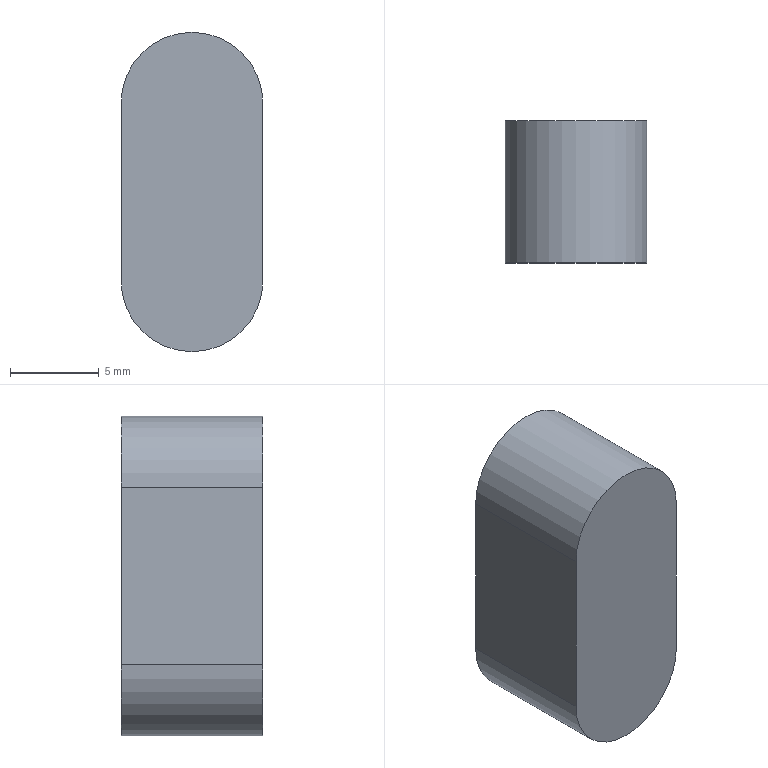Component | NX | FLAT_KEY_3 | 1 solid | 6 faces | box 8 x 8 x 18 mm | volume 1042 mm3 | plane 4 | cylinder 2 | commonest cylinder face diameters 8 x2
STEP:
#1=CARTESIAN_POINT('',(0.,0.,0.));
#2=DIRECTION('',(0.,0.,1.));
#3=DIRECTION('',(1.,0.,0.));
#4=AXIS2_PLACEMENT_3D('',#1,#2,#3);
#5=CARTESIAN_POINT('',(-602.175,316.681,-695.));
#6=VERTEX_POINT('',#5);
#7=CARTESIAN_POINT('',(-602.175,316.681,-685.));
#8=VERTEX_POINT('',#7);
#9=CARTESIAN_POINT('',(-602.175,316.681,-690.));
#10=DIRECTION('',(0.,0.,1.));
#11=VECTOR('',#10,1.);
#12=LINE('',#9,#11);
#13=CARTESIAN_POINT('',(-598.175,316.681,-690.));
#14=DIRECTION('',(0.,-1.,0.));
#15=DIRECTION('',(0.,0.,-1.));
#16=AXIS2_PLACEMENT_3D('',#13,#14,#15);
#17=PLANE('',#16);
#18=CARTESIAN_POINT('',(0.,-4.));
#19=DIRECTION('',(-1.,0.));
#20=VECTOR('',#19,1.);
#21=LINE('',#18,#20);
#22=(GEOMETRIC_REPRESENTATION_CONTEXT(2)PARAMETRIC_REPRESENTATION_CONTEXT()REPRESENTATION_CONTEXT('',''));
#23=DEFINITIONAL_REPRESENTATION('',(#21),#22);
#24=PCURVE('',#17,#23);
#25=CARTESIAN_POINT('',(-602.175,324.681,-690.));
#26=DIRECTION('',(-1.,0.,0.));
#27=DIRECTION('',(0.,1.,0.));
#28=AXIS2_PLACEMENT_3D('',#25,#26,#27);
#29=PLANE('',#28);
#30=CARTESIAN_POINT('',(-8.,0.));
#31=DIRECTION('',(0.,-1.));
#32=VECTOR('',#31,1.);
#33=LINE('',#30,#32);
#34=(GEOMETRIC_REPRESENTATION_CONTEXT(2)PARAMETRIC_REPRESENTATION_CONTEXT()REPRESENTATION_CONTEXT('',''));
#35=DEFINITIONAL_REPRESENTATION('',(#33),#34);
#36=PCURVE('',#29,#35);
#37=SURFACE_CURVE('',#12,(#24,#36),.PCURVE_S1.);
#38=EDGE_CURVE('',#6,#8,#37,.T.);
#39=ORIENTED_EDGE('',*,*,#38,.F.);
#40=CARTESIAN_POINT('',(-594.175,316.681,-695.));
#41=VERTEX_POINT('',#40);
#42=CARTESIAN_POINT('',(-598.175,316.681,-695.));
#43=DIRECTION('',(0.,-1.,0.));
#44=DIRECTION('',(0.,0.,-1.));
#45=AXIS2_PLACEMENT_3D('',#42,#43,#44);
#46=CIRCLE('',#45,4.);
#47=CARTESIAN_POINT('',(5.,0.));
#48=DIRECTION('',(1.,0.));
#49=AXIS2_PLACEMENT_2D('',#47,#48);
#50=CIRCLE('',#49,4.);
#51=(GEOMETRIC_REPRESENTATION_CONTEXT(2)PARAMETRIC_REPRESENTATION_CONTEXT()REPRESENTATION_CONTEXT('',''));
#52=DEFINITIONAL_REPRESENTATION('',(#50),#51);
#53=PCURVE('',#17,#52);
#54=CARTESIAN_POINT('',(-598.175,324.681,-695.));
#55=DIRECTION('',(0.,-1.,0.));
#56=DIRECTION('',(0.,0.,-1.));
#57=AXIS2_PLACEMENT_3D('',#54,#55,#56);
#58=CYLINDRICAL_SURFACE('',#57,4.);
#59=CARTESIAN_POINT('',(0.,8.));
#60=DIRECTION('',(1.,0.));
#61=VECTOR('',#60,1.);
#62=LINE('',#59,#61);
#63=(GEOMETRIC_REPRESENTATION_CONTEXT(2)PARAMETRIC_REPRESENTATION_CONTEXT()REPRESENTATION_CONTEXT('',''));
#64=DEFINITIONAL_REPRESENTATION('',(#62),#63);
#65=PCURVE('',#58,#64);
#66=SURFACE_CURVE('',#46,(#53,#65),.PCURVE_S1.);
#67=EDGE_CURVE('',#6,#41,#66,.T.);
#68=ORIENTED_EDGE('',*,*,#67,.T.);
#69=CARTESIAN_POINT('',(-594.175,316.681,-685.));
#70=VERTEX_POINT('',#69);
#71=CARTESIAN_POINT('',(-594.175,316.681,-690.));
#72=DIRECTION('',(0.,0.,-1.));
#73=VECTOR('',#72,1.);
#74=LINE('',#71,#73);
#75=CARTESIAN_POINT('',(0.,4.));
#76=DIRECTION('',(1.,0.));
#77=VECTOR('',#76,1.);
#78=LINE('',#75,#77);
#79=(GEOMETRIC_REPRESENTATION_CONTEXT(2)PARAMETRIC_REPRESENTATION_CONTEXT()REPRESENTATION_CONTEXT('',''));
#80=DEFINITIONAL_REPRESENTATION('',(#78),#79);
#81=PCURVE('',#17,#80);
#82=CARTESIAN_POINT('',(-594.175,324.681,-690.));
#83=DIRECTION('',(1.,0.,0.));
#84=DIRECTION('',(0.,-1.,0.));
#85=AXIS2_PLACEMENT_3D('',#82,#83,#84);
#86=PLANE('',#85);
#87=CARTESIAN_POINT('',(8.,0.));
#88=DIRECTION('',(0.,1.));
#89=VECTOR('',#88,1.);
#90=LINE('',#87,#89);
#91=(GEOMETRIC_REPRESENTATION_CONTEXT(2)PARAMETRIC_REPRESENTATION_CONTEXT()REPRESENTATION_CONTEXT('',''));
#92=DEFINITIONAL_REPRESENTATION('',(#90),#91);
#93=PCURVE('',#86,#92);
#94=SURFACE_CURVE('',#74,(#81,#93),.PCURVE_S1.);
#95=EDGE_CURVE('',#70,#41,#94,.T.);
#96=ORIENTED_EDGE('',*,*,#95,.F.);
#97=CARTESIAN_POINT('',(-598.175,316.681,-685.));
#98=DIRECTION('',(0.,-1.,0.));
#99=DIRECTION('',(0.,0.,-1.));
#100=AXIS2_PLACEMENT_3D('',#97,#98,#99);
#101=CIRCLE('',#100,4.);
#102=CARTESIAN_POINT('',(-5.,0.));
#103=DIRECTION('',(1.,0.));
#104=AXIS2_PLACEMENT_2D('',#102,#103);
#105=CIRCLE('',#104,4.);
#106=(GEOMETRIC_REPRESENTATION_CONTEXT(2)PARAMETRIC_REPRESENTATION_CONTEXT()REPRESENTATION_CONTEXT('',''));
#107=DEFINITIONAL_REPRESENTATION('',(#105),#106);
#108=PCURVE('',#17,#107);
#109=CARTESIAN_POINT('',(-598.175,324.681,-685.));
#110=DIRECTION('',(0.,-1.,0.));
#111=DIRECTION('',(0.,0.,-1.));
#112=AXIS2_PLACEMENT_3D('',#109,#110,#111);
#113=CYLINDRICAL_SURFACE('',#112,4.);
#114=CARTESIAN_POINT('',(0.,8.));
#115=DIRECTION('',(1.,0.));
#116=VECTOR('',#115,1.);
#117=LINE('',#114,#116);
#118=(GEOMETRIC_REPRESENTATION_CONTEXT(2)PARAMETRIC_REPRESENTATION_CONTEXT()REPRESENTATION_CONTEXT('',''));
#119=DEFINITIONAL_REPRESENTATION('',(#117),#118);
#120=PCURVE('',#113,#119);
#121=SURFACE_CURVE('',#101,(#108,#120),.PCURVE_S1.);
#122=EDGE_CURVE('',#70,#8,#121,.T.);
#123=ORIENTED_EDGE('',*,*,#122,.T.);
#124=EDGE_LOOP('',(#39,#68,#96,#123));
#125=FACE_BOUND('',#124,.T.);
#126=ADVANCED_FACE('',(#125),#17,.T.);
#127=CARTESIAN_POINT('',(-602.175,324.681,-685.));
#128=VERTEX_POINT('',#127);
#129=CARTESIAN_POINT('',(-602.175,324.681,-695.));
#130=VERTEX_POINT('',#129);
#131=CARTESIAN_POINT('',(-602.175,324.681,-690.));
#132=DIRECTION('',(0.,0.,-1.));
#133=VECTOR('',#132,1.);
#134=LINE('',#131,#133);
#135=CARTESIAN_POINT('',(0.,0.));
#136=DIRECTION('',(0.,1.));
#137=VECTOR('',#136,1.);
#138=LINE('',#135,#137);
#139=(GEOMETRIC_REPRESENTATION_CONTEXT(2)PARAMETRIC_REPRESENTATION_CONTEXT()REPRESENTATION_CONTEXT('',''));
#140=DEFINITIONAL_REPRESENTATION('',(#138),#139);
#141=PCURVE('',#29,#140);
#142=CARTESIAN_POINT('',(-598.175,324.681,-690.));
#143=DIRECTION('',(0.,1.,0.));
#144=DIRECTION('',(0.,0.,1.));
#145=AXIS2_PLACEMENT_3D('',#142,#143,#144);
#146=PLANE('',#145);
#147=CARTESIAN_POINT('',(0.,-4.));
#148=DIRECTION('',(-1.,0.));
#149=VECTOR('',#148,1.);
#150=LINE('',#147,#149);
#151=(GEOMETRIC_REPRESENTATION_CONTEXT(2)PARAMETRIC_REPRESENTATION_CONTEXT()REPRESENTATION_CONTEXT('',''));
#152=DEFINITIONAL_REPRESENTATION('',(#150),#151);
#153=PCURVE('',#146,#152);
#154=SURFACE_CURVE('',#134,(#141,#153),.PCURVE_S1.);
#155=EDGE_CURVE('',#128,#130,#154,.T.);
#156=ORIENTED_EDGE('',*,*,#155,.T.);
#157=CARTESIAN_POINT('',(-602.175,324.681,-695.));
#158=DIRECTION('',(0.,-1.,0.));
#159=VECTOR('',#158,1.);
#160=LINE('',#157,#159);
#161=CARTESIAN_POINT('',(0.,5.));
#162=DIRECTION('',(-1.,0.));
#163=VECTOR('',#162,1.);
#164=LINE('',#161,#163);
#165=(GEOMETRIC_REPRESENTATION_CONTEXT(2)PARAMETRIC_REPRESENTATION_CONTEXT()REPRESENTATION_CONTEXT('',''));
#166=DEFINITIONAL_REPRESENTATION('',(#164),#165);
#167=PCURVE('',#29,#166);
#168=CARTESIAN_POINT('',(4.712,0.));
#169=DIRECTION('',(0.,1.));
#170=VECTOR('',#169,1.);
#171=LINE('',#168,#170);
#172=(GEOMETRIC_REPRESENTATION_CONTEXT(2)PARAMETRIC_REPRESENTATION_CONTEXT()REPRESENTATION_CONTEXT('',''));
#173=DEFINITIONAL_REPRESENTATION('',(#171),#172);
#174=PCURVE('',#58,#173);
#175=SURFACE_CURVE('',#160,(#167,#174),.PCURVE_S1.);
#176=EDGE_CURVE('',#130,#6,#175,.T.);
#177=ORIENTED_EDGE('',*,*,#176,.T.);
#178=ORIENTED_EDGE('',*,*,#38,.T.);
#179=CARTESIAN_POINT('',(-602.175,324.681,-685.));
#180=DIRECTION('',(0.,1.,0.));
#181=VECTOR('',#180,1.);
#182=LINE('',#179,#181);
#183=CARTESIAN_POINT('',(0.,-5.));
#184=DIRECTION('',(1.,0.));
#185=VECTOR('',#184,1.);
#186=LINE('',#183,#185);
#187=(GEOMETRIC_REPRESENTATION_CONTEXT(2)PARAMETRIC_REPRESENTATION_CONTEXT()REPRESENTATION_CONTEXT('',''));
#188=DEFINITIONAL_REPRESENTATION('',(#186),#187);
#189=PCURVE('',#29,#188);
#190=CARTESIAN_POINT('',(4.712,0.));
#191=DIRECTION('',(0.,-1.));
#192=VECTOR('',#191,1.);
#193=LINE('',#190,#192);
#194=(GEOMETRIC_REPRESENTATION_CONTEXT(2)PARAMETRIC_REPRESENTATION_CONTEXT()REPRESENTATION_CONTEXT('',''));
#195=DEFINITIONAL_REPRESENTATION('',(#193),#194);
#196=PCURVE('',#113,#195);
#197=SURFACE_CURVE('',#182,(#189,#196),.PCURVE_S1.);
#198=EDGE_CURVE('',#8,#128,#197,.T.);
#199=ORIENTED_EDGE('',*,*,#198,.T.);
#200=EDGE_LOOP('',(#156,#177,#178,#199));
#201=FACE_BOUND('',#200,.T.);
#202=ADVANCED_FACE('',(#201),#29,.T.);
#203=ORIENTED_EDGE('',*,*,#95,.T.);
#204=CARTESIAN_POINT('',(-594.175,324.681,-695.));
#205=VERTEX_POINT('',#204);
#206=CARTESIAN_POINT('',(-594.175,324.681,-695.));
#207=DIRECTION('',(0.,1.,0.));
#208=VECTOR('',#207,1.);
#209=LINE('',#206,#208);
#210=CARTESIAN_POINT('',(0.,5.));
#211=DIRECTION('',(-1.,0.));
#212=VECTOR('',#211,1.);
#213=LINE('',#210,#212);
#214=(GEOMETRIC_REPRESENTATION_CONTEXT(2)PARAMETRIC_REPRESENTATION_CONTEXT()REPRESENTATION_CONTEXT('',''));
#215=DEFINITIONAL_REPRESENTATION('',(#213),#214);
#216=PCURVE('',#86,#215);
#217=CARTESIAN_POINT('',(7.854,0.));
#218=DIRECTION('',(0.,-1.));
#219=VECTOR('',#218,1.);
#220=LINE('',#217,#219);
#221=(GEOMETRIC_REPRESENTATION_CONTEXT(2)PARAMETRIC_REPRESENTATION_CONTEXT()REPRESENTATION_CONTEXT('',''));
#222=DEFINITIONAL_REPRESENTATION('',(#220),#221);
#223=PCURVE('',#58,#222);
#224=SURFACE_CURVE('',#209,(#216,#223),.PCURVE_S1.);
#225=EDGE_CURVE('',#41,#205,#224,.T.);
#226=ORIENTED_EDGE('',*,*,#225,.T.);
#227=CARTESIAN_POINT('',(-594.175,324.681,-685.));
#228=VERTEX_POINT('',#227);
#229=CARTESIAN_POINT('',(-594.175,324.681,-690.));
#230=DIRECTION('',(0.,0.,1.));
#231=VECTOR('',#230,1.);
#232=LINE('',#229,#231);
#233=CARTESIAN_POINT('',(0.,0.));
#234=DIRECTION('',(0.,-1.));
#235=VECTOR('',#234,1.);
#236=LINE('',#233,#235);
#237=(GEOMETRIC_REPRESENTATION_CONTEXT(2)PARAMETRIC_REPRESENTATION_CONTEXT()REPRESENTATION_CONTEXT('',''));
#238=DEFINITIONAL_REPRESENTATION('',(#236),#237);
#239=PCURVE('',#86,#238);
#240=CARTESIAN_POINT('',(0.,4.));
#241=DIRECTION('',(1.,0.));
#242=VECTOR('',#241,1.);
#243=LINE('',#240,#242);
#244=(GEOMETRIC_REPRESENTATION_CONTEXT(2)PARAMETRIC_REPRESENTATION_CONTEXT()REPRESENTATION_CONTEXT('',''));
#245=DEFINITIONAL_REPRESENTATION('',(#243),#244);
#246=PCURVE('',#146,#245);
#247=SURFACE_CURVE('',#232,(#239,#246),.PCURVE_S1.);
#248=EDGE_CURVE('',#205,#228,#247,.T.);
#249=ORIENTED_EDGE('',*,*,#248,.T.);
#250=CARTESIAN_POINT('',(-594.175,324.681,-685.));
#251=DIRECTION('',(0.,-1.,0.));
#252=VECTOR('',#251,1.);
#253=LINE('',#250,#252);
#254=CARTESIAN_POINT('',(0.,-5.));
#255=DIRECTION('',(1.,0.));
#256=VECTOR('',#255,1.);
#257=LINE('',#254,#256);
#258=(GEOMETRIC_REPRESENTATION_CONTEXT(2)PARAMETRIC_REPRESENTATION_CONTEXT()REPRESENTATION_CONTEXT('',''));
#259=DEFINITIONAL_REPRESENTATION('',(#257),#258);
#260=PCURVE('',#86,#259);
#261=CARTESIAN_POINT('',(1.571,0.));
#262=DIRECTION('',(0.,1.));
#263=VECTOR('',#262,1.);
#264=LINE('',#261,#263);
#265=(GEOMETRIC_REPRESENTATION_CONTEXT(2)PARAMETRIC_REPRESENTATION_CONTEXT()REPRESENTATION_CONTEXT('',''));
#266=DEFINITIONAL_REPRESENTATION('',(#264),#265);
#267=PCURVE('',#113,#266);
#268=SURFACE_CURVE('',#253,(#260,#267),.PCURVE_S1.);
#269=EDGE_CURVE('',#228,#70,#268,.T.);
#270=ORIENTED_EDGE('',*,*,#269,.T.);
#271=EDGE_LOOP('',(#203,#226,#249,#270));
#272=FACE_BOUND('',#271,.T.);
#273=ADVANCED_FACE('',(#272),#86,.T.);
#274=CARTESIAN_POINT('',(-598.175,324.681,-695.));
#275=DIRECTION('',(0.,1.,0.));
#276=DIRECTION('',(0.,0.,1.));
#277=AXIS2_PLACEMENT_3D('',#274,#275,#276);
#278=CIRCLE('',#277,4.);
#279=CARTESIAN_POINT('',(-5.,0.));
#280=DIRECTION('',(1.,0.));
#281=AXIS2_PLACEMENT_2D('',#279,#280);
#282=CIRCLE('',#281,4.);
#283=(GEOMETRIC_REPRESENTATION_CONTEXT(2)PARAMETRIC_REPRESENTATION_CONTEXT()REPRESENTATION_CONTEXT('',''));
#284=DEFINITIONAL_REPRESENTATION('',(#282),#283);
#285=PCURVE('',#146,#284);
#286=CARTESIAN_POINT('',(9.425,0.));
#287=DIRECTION('',(-1.,0.));
#288=VECTOR('',#287,1.);
#289=LINE('',#286,#288);
#290=(GEOMETRIC_REPRESENTATION_CONTEXT(2)PARAMETRIC_REPRESENTATION_CONTEXT()REPRESENTATION_CONTEXT('',''));
#291=DEFINITIONAL_REPRESENTATION('',(#289),#290);
#292=PCURVE('',#58,#291);
#293=SURFACE_CURVE('',#278,(#285,#292),.PCURVE_S1.);
#294=EDGE_CURVE('',#205,#130,#293,.T.);
#295=ORIENTED_EDGE('',*,*,#294,.T.);
#296=ORIENTED_EDGE('',*,*,#155,.F.);
#297=CARTESIAN_POINT('',(-598.175,324.681,-685.));
#298=DIRECTION('',(0.,1.,0.));
#299=DIRECTION('',(0.,0.,1.));
#300=AXIS2_PLACEMENT_3D('',#297,#298,#299);
#301=CIRCLE('',#300,4.);
#302=CARTESIAN_POINT('',(5.,0.));
#303=DIRECTION('',(1.,0.));
#304=AXIS2_PLACEMENT_2D('',#302,#303);
#305=CIRCLE('',#304,4.);
#306=(GEOMETRIC_REPRESENTATION_CONTEXT(2)PARAMETRIC_REPRESENTATION_CONTEXT()REPRESENTATION_CONTEXT('',''));
#307=DEFINITIONAL_REPRESENTATION('',(#305),#306);
#308=PCURVE('',#146,#307);
#309=CARTESIAN_POINT('',(9.425,0.));
#310=DIRECTION('',(-1.,0.));
#311=VECTOR('',#310,1.);
#312=LINE('',#309,#311);
#313=(GEOMETRIC_REPRESENTATION_CONTEXT(2)PARAMETRIC_REPRESENTATION_CONTEXT()REPRESENTATION_CONTEXT('',''));
#314=DEFINITIONAL_REPRESENTATION('',(#312),#313);
#315=PCURVE('',#113,#314);
#316=SURFACE_CURVE('',#301,(#308,#315),.PCURVE_S1.);
#317=EDGE_CURVE('',#128,#228,#316,.T.);
#318=ORIENTED_EDGE('',*,*,#317,.T.);
#319=ORIENTED_EDGE('',*,*,#248,.F.);
#320=EDGE_LOOP('',(#295,#296,#318,#319));
#321=FACE_BOUND('',#320,.T.);
#322=ADVANCED_FACE('',(#321),#146,.T.);
#323=ORIENTED_EDGE('',*,*,#67,.F.);
#324=ORIENTED_EDGE('',*,*,#176,.F.);
#325=ORIENTED_EDGE('',*,*,#294,.F.);
#326=ORIENTED_EDGE('',*,*,#225,.F.);
#327=EDGE_LOOP('',(#323,#324,#325,#326));
#328=FACE_BOUND('',#327,.T.);
#329=ADVANCED_FACE('',(#328),#58,.T.);
#330=ORIENTED_EDGE('',*,*,#122,.F.);
#331=ORIENTED_EDGE('',*,*,#269,.F.);
#332=ORIENTED_EDGE('',*,*,#317,.F.);
#333=ORIENTED_EDGE('',*,*,#198,.F.);
#334=EDGE_LOOP('',(#330,#331,#332,#333));
#335=FACE_BOUND('',#334,.T.);
#336=ADVANCED_FACE('',(#335),#113,.T.);
#337=CLOSED_SHELL('',(#126,#202,#273,#322,#329,#336));
#338=MANIFOLD_SOLID_BREP('',#337);
#339=(LENGTH_UNIT()NAMED_UNIT(*)SI_UNIT(.MILLI.,.METRE.));
#340=UNCERTAINTY_MEASURE_WITH_UNIT(LENGTH_MEASURE(0.0000001),#339,'','');
#341=(NAMED_UNIT(*)PLANE_ANGLE_UNIT()SI_UNIT($,.RADIAN.));
#342=(NAMED_UNIT(*)SI_UNIT($,.STERADIAN.)SOLID_ANGLE_UNIT());
#343=(GEOMETRIC_REPRESENTATION_CONTEXT(3)GLOBAL_UNCERTAINTY_ASSIGNED_CONTEXT((#340))GLOBAL_UNIT_ASSIGNED_CONTEXT((#339,#341,#342))REPRESENTATION_CONTEXT('',''));
#344=ADVANCED_BREP_SHAPE_REPRESENTATION('',(#4,#338),#343);